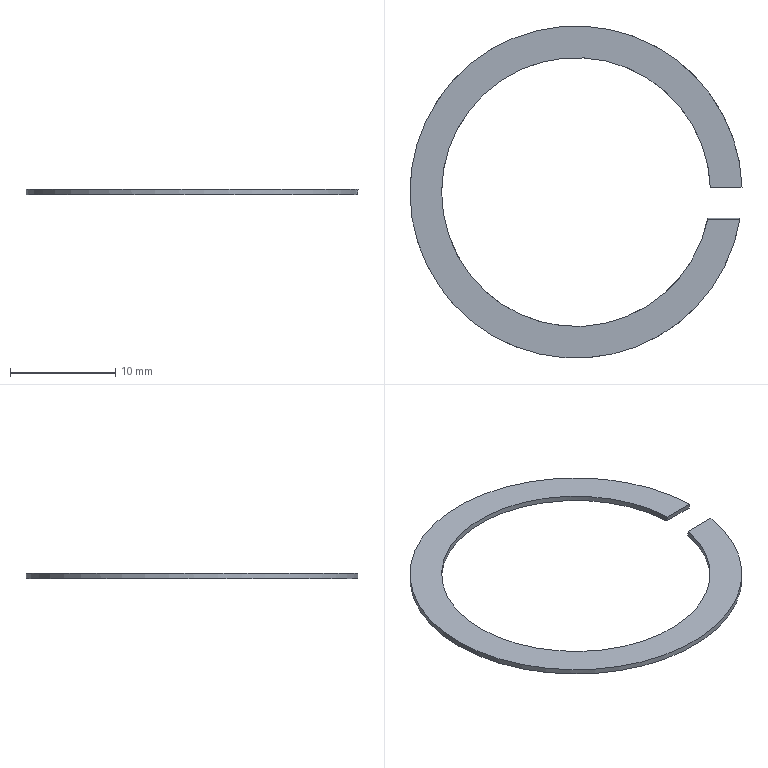Component | NX | GASKET | 1 solid | 6 faces | box 31.49 x 31.5 x 0.5 mm | volume 130 mm3 | plane 4 | cylinder 2 | commonest cylinder face diameters 31.5 x1 25.5 x1
STEP:
#1=CARTESIAN_POINT('',(0.,0.,0.));
#2=DIRECTION('',(0.,0.,1.));
#3=DIRECTION('',(1.,0.,0.));
#4=AXIS2_PLACEMENT_3D('',#1,#2,#3);
#5=CARTESIAN_POINT('',(15.551,-2.493,-0.5));
#6=VERTEX_POINT('',#5);
#7=CARTESIAN_POINT('',(15.74,0.5533,-0.5));
#8=VERTEX_POINT('',#7);
#9=CARTESIAN_POINT('',(0.,0.,-0.5));
#10=DIRECTION('',(0.,0.,-1.));
#11=DIRECTION('',(-1.,0.,0.));
#12=AXIS2_PLACEMENT_3D('',#9,#10,#11);
#13=CIRCLE('',#12,15.75);
#14=CARTESIAN_POINT('',(0.,0.,-6.));
#15=DIRECTION('',(0.,0.,-1.));
#16=DIRECTION('',(-1.,0.,0.));
#17=AXIS2_PLACEMENT_3D('',#14,#15,#16);
#18=CYLINDRICAL_SURFACE('',#17,15.75);
#19=CARTESIAN_POINT('',(-6.283,-5.5));
#20=DIRECTION('',(1.,0.));
#21=VECTOR('',#20,1.);
#22=LINE('',#19,#21);
#23=(GEOMETRIC_REPRESENTATION_CONTEXT(2)PARAMETRIC_REPRESENTATION_CONTEXT()REPRESENTATION_CONTEXT('',''));
#24=DEFINITIONAL_REPRESENTATION('',(#22),#23);
#25=PCURVE('',#18,#24);
#26=CARTESIAN_POINT('',(0.,12.75,-0.5));
#27=DIRECTION('',(0.,0.,-1.));
#28=DIRECTION('',(-1.,0.,0.));
#29=AXIS2_PLACEMENT_3D('',#26,#27,#28);
#30=PLANE('',#29);
#31=CARTESIAN_POINT('',(0.,-12.75));
#32=DIRECTION('',(1.,0.));
#33=AXIS2_PLACEMENT_2D('',#31,#32);
#34=CIRCLE('',#33,15.75);
#35=(GEOMETRIC_REPRESENTATION_CONTEXT(2)PARAMETRIC_REPRESENTATION_CONTEXT()REPRESENTATION_CONTEXT('',''));
#36=DEFINITIONAL_REPRESENTATION('',(#34),#35);
#37=PCURVE('',#30,#36);
#38=SURFACE_CURVE('',#13,(#25,#37),.PCURVE_S1.);
#39=EDGE_CURVE('',#6,#8,#38,.T.);
#40=ORIENTED_EDGE('',*,*,#39,.F.);
#41=CARTESIAN_POINT('',(15.537,-2.581,0.));
#42=VERTEX_POINT('',#41);
#43=CARTESIAN_POINT('',(0.,0.,-14.638));
#44=DIRECTION('',(0.,-0.9848,-0.1736));
#45=DIRECTION('',(0.,0.1736,-0.9848));
#46=AXIS2_PLACEMENT_3D('',#43,#44,#45);
#47=ELLIPSE('',#46,90.701,15.75);
#48=CARTESIAN_POINT('',(-2.983,-5.5));
#49=CARTESIAN_POINT('',(-2.977,-6.));
#50=B_SPLINE_CURVE_WITH_KNOTS('',1,(#48,#49),.UNSPECIFIED.,.F.,.F.,(2,2),(1.73,1.735),.PIECEWISE_BEZIER_KNOTS.);
#51=(GEOMETRIC_REPRESENTATION_CONTEXT(2)PARAMETRIC_REPRESENTATION_CONTEXT()REPRESENTATION_CONTEXT('',''));
#52=DEFINITIONAL_REPRESENTATION('',(#50),#51);
#53=PCURVE('',#18,#52);
#54=CARTESIAN_POINT('',(28.125,-3.04,2.603));
#55=DIRECTION('',(0.,0.9848,0.1736));
#56=DIRECTION('',(0.,-0.1736,0.9848));
#57=AXIS2_PLACEMENT_3D('',#54,#55,#56);
#58=PLANE('',#57);
#59=CARTESIAN_POINT('',(-108.208,-28.125));
#60=CARTESIAN_POINT('',(-108.208,-0.8452));
#61=CARTESIAN_POINT('',(27.843,-14.485));
#62=CARTESIAN_POINT('',(163.894,-28.125));
#63=CARTESIAN_POINT('',(27.843,-41.765));
#64=CARTESIAN_POINT('',(-108.208,-55.405));
#65=CARTESIAN_POINT('',(-108.208,-28.125));
#66=(BOUNDED_CURVE()B_SPLINE_CURVE(2,(#59,#60,#61,#62,#63,#64,#65),.UNSPECIFIED.,.T.,.F.)B_SPLINE_CURVE_WITH_KNOTS((1,2,2,2,2,1),(-2.094,0.,2.094,4.189,6.283,8.378),.UNSPECIFIED.)CURVE()GEOMETRIC_REPRESENTATION_ITEM()RATIONAL_B_SPLINE_CURVE((1.,0.5,1.,0.5,1.,0.5,1.))REPRESENTATION_ITEM(''));
#67=(GEOMETRIC_REPRESENTATION_CONTEXT(2)PARAMETRIC_REPRESENTATION_CONTEXT()REPRESENTATION_CONTEXT('',''));
#68=DEFINITIONAL_REPRESENTATION('',(#66),#67);
#69=PCURVE('',#58,#68);
#70=SURFACE_CURVE('',#47,(#53,#69),.PCURVE_S1.);
#71=EDGE_CURVE('',#6,#42,#70,.T.);
#72=ORIENTED_EDGE('',*,*,#71,.T.);
#73=CARTESIAN_POINT('',(15.743,0.4652,0.));
#74=VERTEX_POINT('',#73);
#75=CARTESIAN_POINT('',(0.,0.,0.));
#76=DIRECTION('',(0.,0.,-1.));
#77=DIRECTION('',(1.,0.,0.));
#78=AXIS2_PLACEMENT_3D('',#75,#76,#77);
#79=CIRCLE('',#78,15.75);
#80=CARTESIAN_POINT('',(-3.142,-6.));
#81=DIRECTION('',(1.,0.));
#82=VECTOR('',#81,1.);
#83=LINE('',#80,#82);
#84=(GEOMETRIC_REPRESENTATION_CONTEXT(2)PARAMETRIC_REPRESENTATION_CONTEXT()REPRESENTATION_CONTEXT('',''));
#85=DEFINITIONAL_REPRESENTATION('',(#83),#84);
#86=PCURVE('',#18,#85);
#87=CARTESIAN_POINT('',(0.,18.75,0.));
#88=DIRECTION('',(0.,0.,1.));
#89=DIRECTION('',(1.,0.,0.));
#90=AXIS2_PLACEMENT_3D('',#87,#88,#89);
#91=PLANE('',#90);
#92=CARTESIAN_POINT('',(15.75,-18.75));
#93=CARTESIAN_POINT('',(15.75,-46.03));
#94=CARTESIAN_POINT('',(-7.875,-32.39));
#95=CARTESIAN_POINT('',(-31.5,-18.75));
#96=CARTESIAN_POINT('',(-7.875,-5.11));
#97=CARTESIAN_POINT('',(15.75,8.53));
#98=CARTESIAN_POINT('',(15.75,-18.75));
#99=(BOUNDED_CURVE()B_SPLINE_CURVE(2,(#92,#93,#94,#95,#96,#97,#98),.UNSPECIFIED.,.T.,.F.)B_SPLINE_CURVE_WITH_KNOTS((1,2,2,2,2,1),(-2.094,0.,2.094,4.189,6.283,8.378),.UNSPECIFIED.)CURVE()GEOMETRIC_REPRESENTATION_ITEM()RATIONAL_B_SPLINE_CURVE((1.,0.5,1.,0.5,1.,0.5,1.))REPRESENTATION_ITEM(''));
#100=(GEOMETRIC_REPRESENTATION_CONTEXT(2)PARAMETRIC_REPRESENTATION_CONTEXT()REPRESENTATION_CONTEXT('',''));
#101=DEFINITIONAL_REPRESENTATION('',(#99),#100);
#102=PCURVE('',#91,#101);
#103=SURFACE_CURVE('',#79,(#86,#102),.PCURVE_S1.);
#104=EDGE_CURVE('',#42,#74,#103,.T.);
#105=ORIENTED_EDGE('',*,*,#104,.T.);
#106=CARTESIAN_POINT('',(0.,0.,2.638));
#107=DIRECTION('',(0.,0.9848,0.1736));
#108=DIRECTION('',(0.,0.1736,-0.9848));
#109=AXIS2_PLACEMENT_3D('',#106,#107,#108);
#110=ELLIPSE('',#109,90.701,15.75);
#111=CARTESIAN_POINT('',(3.112,-6.));
#112=CARTESIAN_POINT('',(3.106,-5.5));
#113=B_SPLINE_CURVE_WITH_KNOTS('',1,(#111,#112),.UNSPECIFIED.,.F.,.F.,(2,2),(4.742,4.748),.PIECEWISE_BEZIER_KNOTS.);
#114=(GEOMETRIC_REPRESENTATION_CONTEXT(2)PARAMETRIC_REPRESENTATION_CONTEXT()REPRESENTATION_CONTEXT('',''));
#115=DEFINITIONAL_REPRESENTATION('',(#113),#114);
#116=PCURVE('',#18,#115);
#117=CARTESIAN_POINT('',(28.125,3.04,-14.603));
#118=DIRECTION('',(0.,-0.9848,-0.1736));
#119=DIRECTION('',(0.,0.1736,-0.9848));
#120=AXIS2_PLACEMENT_3D('',#117,#118,#119);
#121=PLANE('',#120);
#122=CARTESIAN_POINT('',(73.194,-28.125));
#123=CARTESIAN_POINT('',(73.194,-55.405));
#124=CARTESIAN_POINT('',(-62.857,-41.765));
#125=CARTESIAN_POINT('',(-198.908,-28.125));
#126=CARTESIAN_POINT('',(-62.857,-14.485));
#127=CARTESIAN_POINT('',(73.194,-0.8452));
#128=CARTESIAN_POINT('',(73.194,-28.125));
#129=(BOUNDED_CURVE()B_SPLINE_CURVE(2,(#122,#123,#124,#125,#126,#127,#128),.UNSPECIFIED.,.T.,.F.)B_SPLINE_CURVE_WITH_KNOTS((1,2,2,2,2,1),(-2.094,0.,2.094,4.189,6.283,8.378),.UNSPECIFIED.)CURVE()GEOMETRIC_REPRESENTATION_ITEM()RATIONAL_B_SPLINE_CURVE((1.,0.5,1.,0.5,1.,0.5,1.))REPRESENTATION_ITEM(''));
#130=(GEOMETRIC_REPRESENTATION_CONTEXT(2)PARAMETRIC_REPRESENTATION_CONTEXT()REPRESENTATION_CONTEXT('',''));
#131=DEFINITIONAL_REPRESENTATION('',(#129),#130);
#132=PCURVE('',#121,#131);
#133=SURFACE_CURVE('',#110,(#116,#132),.PCURVE_S1.);
#134=EDGE_CURVE('',#74,#8,#133,.T.);
#135=ORIENTED_EDGE('',*,*,#134,.T.);
#136=EDGE_LOOP('',(#40,#72,#105,#135));
#137=FACE_BOUND('',#136,.T.);
#138=ADVANCED_FACE('',(#137),#18,.T.);
#139=ORIENTED_EDGE('',*,*,#104,.F.);
#140=CARTESIAN_POINT('',(12.486,-2.581,-0.));
#141=VERTEX_POINT('',#140);
#142=CARTESIAN_POINT('',(0.,-2.581,0.));
#143=DIRECTION('',(-1.,0.,0.));
#144=VECTOR('',#143,1.);
#145=LINE('',#142,#144);
#146=CARTESIAN_POINT('',(0.,-21.331));
#147=DIRECTION('',(-1.,0.));
#148=VECTOR('',#147,1.);
#149=LINE('',#146,#148);
#150=(GEOMETRIC_REPRESENTATION_CONTEXT(2)PARAMETRIC_REPRESENTATION_CONTEXT()REPRESENTATION_CONTEXT('',''));
#151=DEFINITIONAL_REPRESENTATION('',(#149),#150);
#152=PCURVE('',#91,#151);
#153=CARTESIAN_POINT('',(-2.643,-28.125));
#154=DIRECTION('',(0.,-1.));
#155=VECTOR('',#154,1.);
#156=LINE('',#153,#155);
#157=(GEOMETRIC_REPRESENTATION_CONTEXT(2)PARAMETRIC_REPRESENTATION_CONTEXT()REPRESENTATION_CONTEXT('',''));
#158=DEFINITIONAL_REPRESENTATION('',(#156),#157);
#159=PCURVE('',#58,#158);
#160=SURFACE_CURVE('',#145,(#152,#159),.PCURVE_S1.);
#161=EDGE_CURVE('',#42,#141,#160,.T.);
#162=ORIENTED_EDGE('',*,*,#161,.T.);
#163=CARTESIAN_POINT('',(12.742,0.4652,0.));
#164=VERTEX_POINT('',#163);
#165=CARTESIAN_POINT('',(0.,0.,0.));
#166=DIRECTION('',(0.,0.,-1.));
#167=DIRECTION('',(-1.,0.,0.));
#168=AXIS2_PLACEMENT_3D('',#165,#166,#167);
#169=CIRCLE('',#168,12.75);
#170=CARTESIAN_POINT('',(-12.75,-18.75));
#171=CARTESIAN_POINT('',(-12.75,3.334));
#172=CARTESIAN_POINT('',(6.375,-7.708));
#173=CARTESIAN_POINT('',(25.5,-18.75));
#174=CARTESIAN_POINT('',(6.375,-29.792));
#175=CARTESIAN_POINT('',(-12.75,-40.834));
#176=CARTESIAN_POINT('',(-12.75,-18.75));
#177=(BOUNDED_CURVE()B_SPLINE_CURVE(2,(#170,#171,#172,#173,#174,#175,#176),.UNSPECIFIED.,.T.,.F.)B_SPLINE_CURVE_WITH_KNOTS((1,2,2,2,2,1),(-2.094,0.,2.094,4.189,6.283,8.378),.UNSPECIFIED.)CURVE()GEOMETRIC_REPRESENTATION_ITEM()RATIONAL_B_SPLINE_CURVE((1.,0.5,1.,0.5,1.,0.5,1.))REPRESENTATION_ITEM(''));
#178=(GEOMETRIC_REPRESENTATION_CONTEXT(2)PARAMETRIC_REPRESENTATION_CONTEXT()REPRESENTATION_CONTEXT('',''));
#179=DEFINITIONAL_REPRESENTATION('',(#177),#178);
#180=PCURVE('',#91,#179);
#181=CARTESIAN_POINT('',(0.,0.,-6.));
#182=DIRECTION('',(0.,0.,-1.));
#183=DIRECTION('',(-1.,0.,0.));
#184=AXIS2_PLACEMENT_3D('',#181,#182,#183);
#185=CYLINDRICAL_SURFACE('',#184,12.75);
#186=CARTESIAN_POINT('',(-6.283,-6.));
#187=DIRECTION('',(1.,0.));
#188=VECTOR('',#187,1.);
#189=LINE('',#186,#188);
#190=(GEOMETRIC_REPRESENTATION_CONTEXT(2)PARAMETRIC_REPRESENTATION_CONTEXT()REPRESENTATION_CONTEXT('',''));
#191=DEFINITIONAL_REPRESENTATION('',(#189),#190);
#192=PCURVE('',#185,#191);
#193=SURFACE_CURVE('',#169,(#180,#192),.PCURVE_S1.);
#194=EDGE_CURVE('',#141,#164,#193,.T.);
#195=ORIENTED_EDGE('',*,*,#194,.T.);
#196=CARTESIAN_POINT('',(0.,0.4652,0.));
#197=DIRECTION('',(1.,0.,0.));
#198=VECTOR('',#197,1.);
#199=LINE('',#196,#198);
#200=CARTESIAN_POINT('',(0.,-18.285));
#201=DIRECTION('',(1.,0.));
#202=VECTOR('',#201,1.);
#203=LINE('',#200,#202);
#204=(GEOMETRIC_REPRESENTATION_CONTEXT(2)PARAMETRIC_REPRESENTATION_CONTEXT()REPRESENTATION_CONTEXT('',''));
#205=DEFINITIONAL_REPRESENTATION('',(#203),#204);
#206=PCURVE('',#91,#205);
#207=CARTESIAN_POINT('',(-14.828,-28.125));
#208=DIRECTION('',(0.,1.));
#209=VECTOR('',#208,1.);
#210=LINE('',#207,#209);
#211=(GEOMETRIC_REPRESENTATION_CONTEXT(2)PARAMETRIC_REPRESENTATION_CONTEXT()REPRESENTATION_CONTEXT('',''));
#212=DEFINITIONAL_REPRESENTATION('',(#210),#211);
#213=PCURVE('',#121,#212);
#214=SURFACE_CURVE('',#199,(#206,#213),.PCURVE_S1.);
#215=EDGE_CURVE('',#164,#74,#214,.T.);
#216=ORIENTED_EDGE('',*,*,#215,.T.);
#217=EDGE_LOOP('',(#139,#162,#195,#216));
#218=FACE_BOUND('',#217,.T.);
#219=ADVANCED_FACE('',(#218),#91,.T.);
#220=CARTESIAN_POINT('',(12.738,0.5533,-0.5));
#221=VERTEX_POINT('',#220);
#222=CARTESIAN_POINT('',(0.,0.,2.638));
#223=DIRECTION('',(0.,-0.9848,-0.1736));
#224=DIRECTION('',(0.,0.1736,-0.9848));
#225=AXIS2_PLACEMENT_3D('',#222,#223,#224);
#226=ELLIPSE('',#225,73.424,12.75);
#227=CARTESIAN_POINT('',(3.098,-5.5));
#228=CARTESIAN_POINT('',(3.105,-6.));
#229=B_SPLINE_CURVE_WITH_KNOTS('',1,(#227,#228),.UNSPECIFIED.,.F.,.F.,(2,2),(1.527,1.534),.PIECEWISE_BEZIER_KNOTS.);
#230=(GEOMETRIC_REPRESENTATION_CONTEXT(2)PARAMETRIC_REPRESENTATION_CONTEXT()REPRESENTATION_CONTEXT('',''));
#231=DEFINITIONAL_REPRESENTATION('',(#229),#230);
#232=PCURVE('',#185,#231);
#233=CARTESIAN_POINT('',(-17.507,-28.125));
#234=DIRECTION('',(1.,0.));
#235=AXIS2_PLACEMENT_2D('',#233,#234);
#236=ELLIPSE('',#235,73.424,12.75);
#237=(GEOMETRIC_REPRESENTATION_CONTEXT(2)PARAMETRIC_REPRESENTATION_CONTEXT()REPRESENTATION_CONTEXT('',''));
#238=DEFINITIONAL_REPRESENTATION('',(#236),#237);
#239=PCURVE('',#121,#238);
#240=SURFACE_CURVE('',#226,(#232,#239),.PCURVE_S1.);
#241=EDGE_CURVE('',#221,#164,#240,.T.);
#242=ORIENTED_EDGE('',*,*,#241,.F.);
#243=CARTESIAN_POINT('',(12.504,-2.493,-0.5));
#244=VERTEX_POINT('',#243);
#245=CARTESIAN_POINT('',(0.,0.,-0.5));
#246=DIRECTION('',(0.,0.,-1.));
#247=DIRECTION('',(-1.,0.,0.));
#248=AXIS2_PLACEMENT_3D('',#245,#246,#247);
#249=CIRCLE('',#248,12.75);
#250=CARTESIAN_POINT('',(-6.283,-5.5));
#251=DIRECTION('',(1.,0.));
#252=VECTOR('',#251,1.);
#253=LINE('',#250,#252);
#254=(GEOMETRIC_REPRESENTATION_CONTEXT(2)PARAMETRIC_REPRESENTATION_CONTEXT()REPRESENTATION_CONTEXT('',''));
#255=DEFINITIONAL_REPRESENTATION('',(#253),#254);
#256=PCURVE('',#185,#255);
#257=CARTESIAN_POINT('',(0.,-12.75));
#258=DIRECTION('',(1.,0.));
#259=AXIS2_PLACEMENT_2D('',#257,#258);
#260=CIRCLE('',#259,12.75);
#261=(GEOMETRIC_REPRESENTATION_CONTEXT(2)PARAMETRIC_REPRESENTATION_CONTEXT()REPRESENTATION_CONTEXT('',''));
#262=DEFINITIONAL_REPRESENTATION('',(#260),#261);
#263=PCURVE('',#30,#262);
#264=SURFACE_CURVE('',#249,(#256,#263),.PCURVE_S1.);
#265=EDGE_CURVE('',#244,#221,#264,.T.);
#266=ORIENTED_EDGE('',*,*,#265,.F.);
#267=CARTESIAN_POINT('',(0.,0.,-14.638));
#268=DIRECTION('',(0.,0.9848,0.1736));
#269=DIRECTION('',(0.,0.1736,-0.9848));
#270=AXIS2_PLACEMENT_3D('',#267,#268,#269);
#271=ELLIPSE('',#270,73.424,12.75);
#272=CARTESIAN_POINT('',(-2.938,-6.));
#273=CARTESIAN_POINT('',(-2.945,-5.5));
#274=B_SPLINE_CURVE_WITH_KNOTS('',1,(#272,#273),.UNSPECIFIED.,.F.,.F.,(2,2),(4.509,4.516),.PIECEWISE_BEZIER_KNOTS.);
#275=(GEOMETRIC_REPRESENTATION_CONTEXT(2)PARAMETRIC_REPRESENTATION_CONTEXT()REPRESENTATION_CONTEXT('',''));
#276=DEFINITIONAL_REPRESENTATION('',(#274),#275);
#277=PCURVE('',#185,#276);
#278=CARTESIAN_POINT('',(-17.507,-28.125));
#279=DIRECTION('',(-1.,0.));
#280=AXIS2_PLACEMENT_2D('',#278,#279);
#281=ELLIPSE('',#280,73.424,12.75);
#282=(GEOMETRIC_REPRESENTATION_CONTEXT(2)PARAMETRIC_REPRESENTATION_CONTEXT()REPRESENTATION_CONTEXT('',''));
#283=DEFINITIONAL_REPRESENTATION('',(#281),#282);
#284=PCURVE('',#58,#283);
#285=SURFACE_CURVE('',#271,(#277,#284),.PCURVE_S1.);
#286=EDGE_CURVE('',#141,#244,#285,.T.);
#287=ORIENTED_EDGE('',*,*,#286,.F.);
#288=ORIENTED_EDGE('',*,*,#194,.T.);
#289=EDGE_LOOP('',(#242,#266,#287,#288));
#290=FACE_BOUND('',#289,.F.);
#291=ADVANCED_FACE('',(#290),#185,.F.);
#292=ORIENTED_EDGE('',*,*,#265,.F.);
#293=CARTESIAN_POINT('',(0.,-2.493,-0.5));
#294=DIRECTION('',(1.,0.,0.));
#295=VECTOR('',#294,1.);
#296=LINE('',#293,#295);
#297=CARTESIAN_POINT('',(0.,-15.243));
#298=DIRECTION('',(-1.,0.));
#299=VECTOR('',#298,1.);
#300=LINE('',#297,#299);
#301=(GEOMETRIC_REPRESENTATION_CONTEXT(2)PARAMETRIC_REPRESENTATION_CONTEXT()REPRESENTATION_CONTEXT('',''));
#302=DEFINITIONAL_REPRESENTATION('',(#300),#301);
#303=PCURVE('',#30,#302);
#304=CARTESIAN_POINT('',(-3.151,-28.125));
#305=DIRECTION('',(0.,1.));
#306=VECTOR('',#305,1.);
#307=LINE('',#304,#306);
#308=(GEOMETRIC_REPRESENTATION_CONTEXT(2)PARAMETRIC_REPRESENTATION_CONTEXT()REPRESENTATION_CONTEXT('',''));
#309=DEFINITIONAL_REPRESENTATION('',(#307),#308);
#310=PCURVE('',#58,#309);
#311=SURFACE_CURVE('',#296,(#303,#310),.PCURVE_S1.);
#312=EDGE_CURVE('',#244,#6,#311,.T.);
#313=ORIENTED_EDGE('',*,*,#312,.T.);
#314=ORIENTED_EDGE('',*,*,#39,.T.);
#315=CARTESIAN_POINT('',(0.,0.5533,-0.5));
#316=DIRECTION('',(-1.,0.,0.));
#317=VECTOR('',#316,1.);
#318=LINE('',#315,#317);
#319=CARTESIAN_POINT('',(0.,-12.197));
#320=DIRECTION('',(1.,0.));
#321=VECTOR('',#320,1.);
#322=LINE('',#319,#321);
#323=(GEOMETRIC_REPRESENTATION_CONTEXT(2)PARAMETRIC_REPRESENTATION_CONTEXT()REPRESENTATION_CONTEXT('',''));
#324=DEFINITIONAL_REPRESENTATION('',(#322),#323);
#325=PCURVE('',#30,#324);
#326=CARTESIAN_POINT('',(-14.32,-28.125));
#327=DIRECTION('',(0.,-1.));
#328=VECTOR('',#327,1.);
#329=LINE('',#326,#328);
#330=(GEOMETRIC_REPRESENTATION_CONTEXT(2)PARAMETRIC_REPRESENTATION_CONTEXT()REPRESENTATION_CONTEXT('',''));
#331=DEFINITIONAL_REPRESENTATION('',(#329),#330);
#332=PCURVE('',#121,#331);
#333=SURFACE_CURVE('',#318,(#325,#332),.PCURVE_S1.);
#334=EDGE_CURVE('',#8,#221,#333,.T.);
#335=ORIENTED_EDGE('',*,*,#334,.T.);
#336=EDGE_LOOP('',(#292,#313,#314,#335));
#337=FACE_BOUND('',#336,.T.);
#338=ADVANCED_FACE('',(#337),#30,.T.);
#339=ORIENTED_EDGE('',*,*,#215,.F.);
#340=ORIENTED_EDGE('',*,*,#241,.F.);
#341=ORIENTED_EDGE('',*,*,#334,.F.);
#342=ORIENTED_EDGE('',*,*,#134,.F.);
#343=EDGE_LOOP('',(#339,#340,#341,#342));
#344=FACE_BOUND('',#343,.T.);
#345=ADVANCED_FACE('',(#344),#121,.T.);
#346=ORIENTED_EDGE('',*,*,#312,.F.);
#347=ORIENTED_EDGE('',*,*,#286,.F.);
#348=ORIENTED_EDGE('',*,*,#161,.F.);
#349=ORIENTED_EDGE('',*,*,#71,.F.);
#350=EDGE_LOOP('',(#346,#347,#348,#349));
#351=FACE_BOUND('',#350,.T.);
#352=ADVANCED_FACE('',(#351),#58,.T.);
#353=CLOSED_SHELL('',(#138,#219,#291,#338,#345,#352));
#354=MANIFOLD_SOLID_BREP('',#353);
#355=(LENGTH_UNIT()NAMED_UNIT(*)SI_UNIT(.MILLI.,.METRE.));
#356=UNCERTAINTY_MEASURE_WITH_UNIT(LENGTH_MEASURE(0.00002),#355,'','');
#357=(NAMED_UNIT(*)PLANE_ANGLE_UNIT()SI_UNIT($,.RADIAN.));
#358=(NAMED_UNIT(*)SI_UNIT($,.STERADIAN.)SOLID_ANGLE_UNIT());
#359=(GEOMETRIC_REPRESENTATION_CONTEXT(3)GLOBAL_UNCERTAINTY_ASSIGNED_CONTEXT((#356))GLOBAL_UNIT_ASSIGNED_CONTEXT((#355,#357,#358))REPRESENTATION_CONTEXT('',''));
#360=ADVANCED_BREP_SHAPE_REPRESENTATION('',(#4,#354),#359);